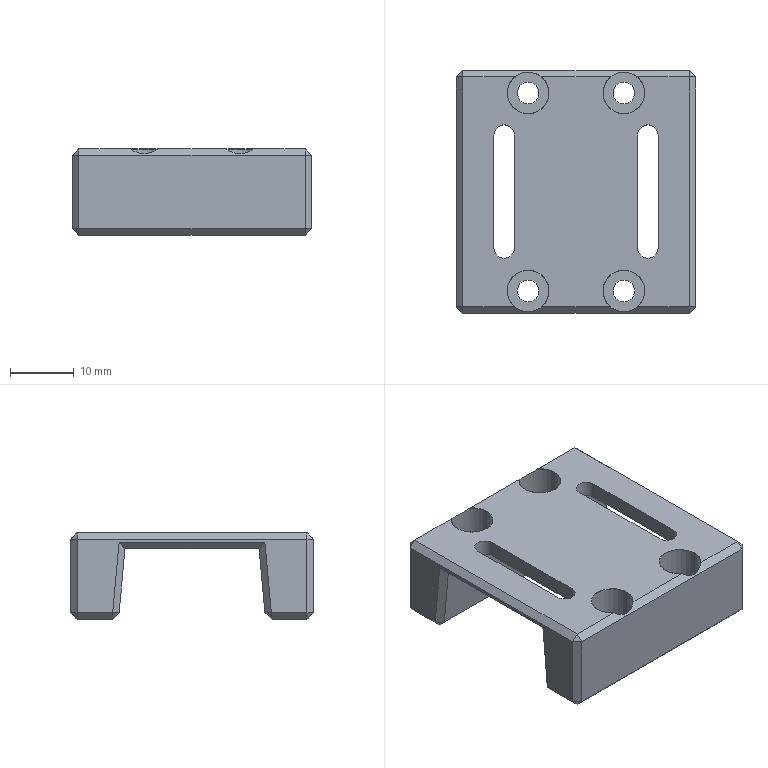CAM job | Mastercam | mm | 16 operations | part box 37.5 x 38 x 13.5
1. Contour (Ramp) | 9 - 10C 平底刀
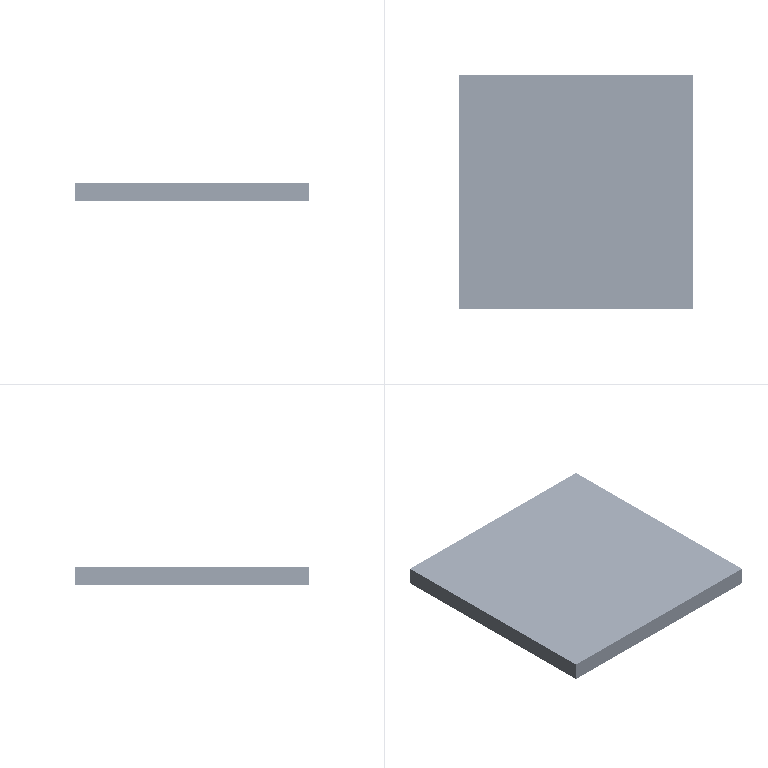2. Facing | 10 - 10J 平底刀
3. 3D High Speed (Dynamic OptiRough) | 6 - 6 平底刀
4. Drill/Counterbore | 2 - 6定位倒角
5. Peck Drill | 12 - 3.4 钻头
6. 3D High Speed (Waterline) | 20 - 4 -R0.5圆鼻铣刀
7. 2D High Speed (2D Blend Mill) | 8 - 6 J平底刀
8. Contour (Ramp) | 13 - 2 平铣刀
9. Contour (2D) | 13 - 2 平铣刀
10. Contour (2D chamfer) | 2 - 6定位倒角
11. Contour (Ramp) | 9 - 10C 平底刀
12. Contour (2D) | 8 - 6 J平底刀
13. Facing | 1 - 50 J面铣
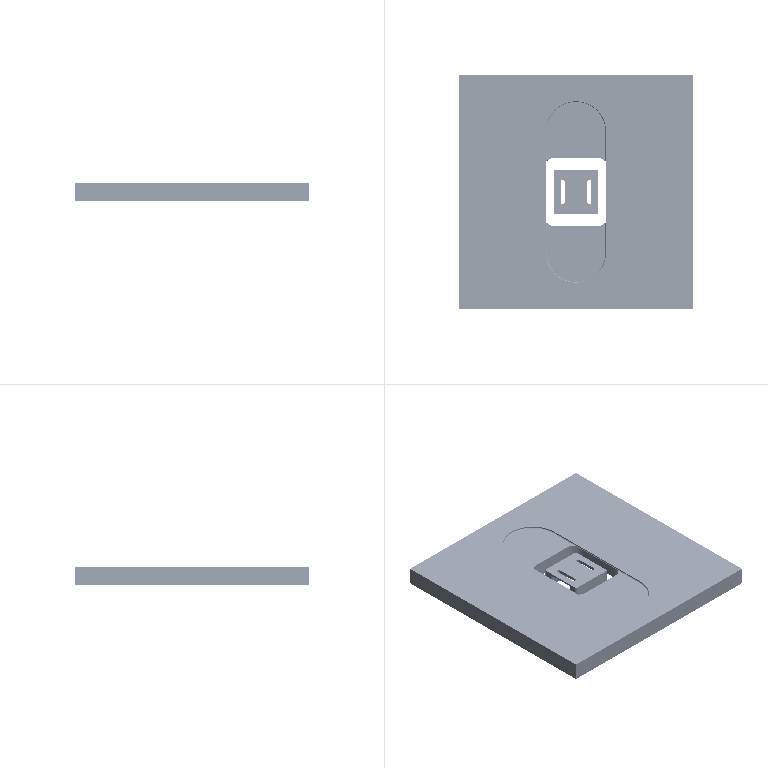14. Helix Bore | 7 - 4 平底刀
15. Contour (2D chamfer) | 2 - 6定位倒角
16. Unified Morph 5axis OP | 20 - 4 -R0.5圆鼻铣刀